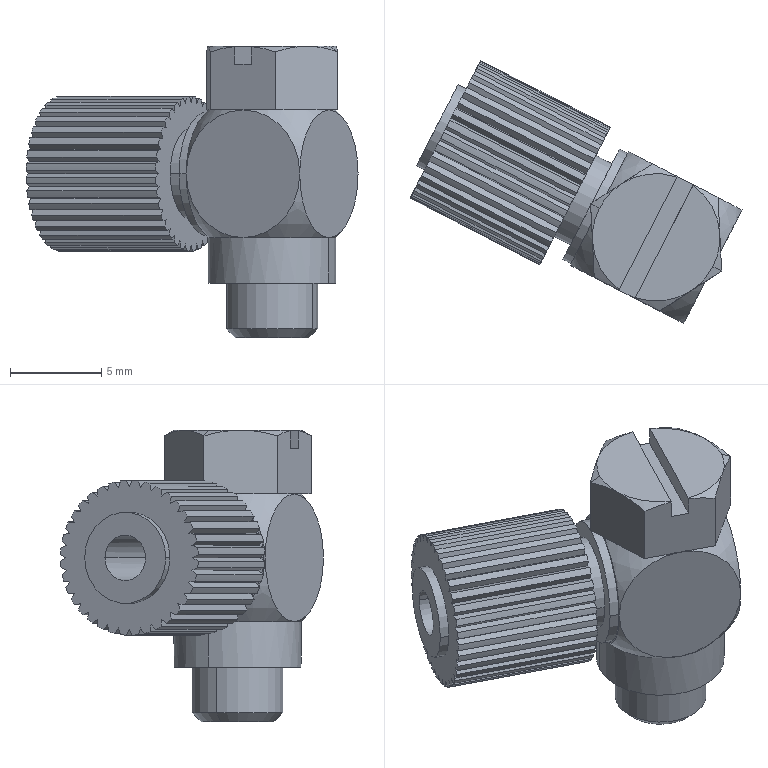Component | SolidWorks | PurchasedPart_MS-5HLH-6StainlessSteelConnector-1 | 1 solid | 181 faces | box 18.22 x 14.43 x 16 mm | volume 995 mm3 | plane 111 | cylinder 54 | cone 10 | sphere 6 | commonest cylinder face diameters 8.5 x36 2.5 x8 5 x6 7 x2 6.8 x2